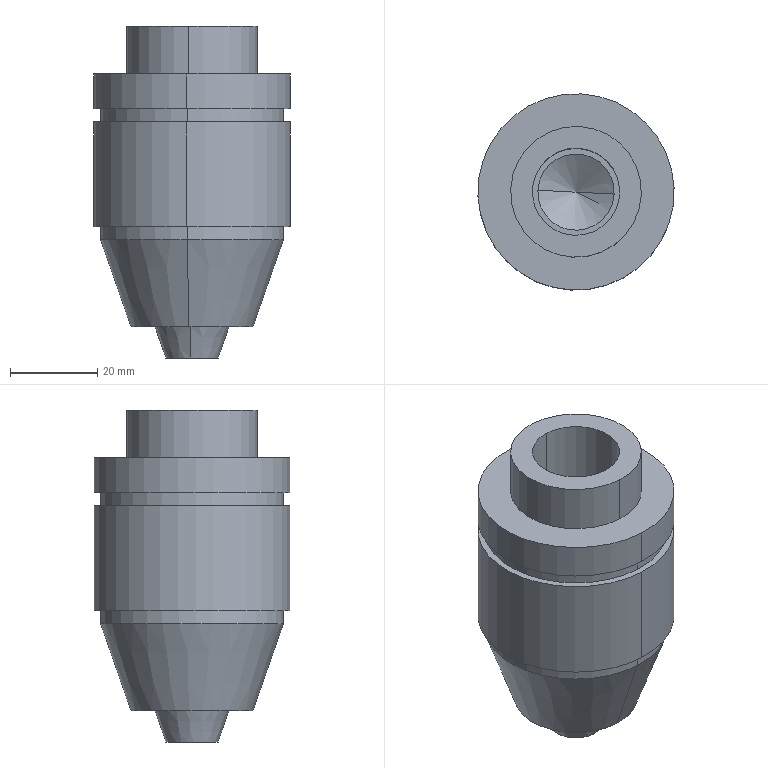Component | SolidWorks | 13-1 | 1 solid | 28 faces | box 45 x 45 x 76.14 mm | volume 73334 mm3 | cylinder 14 | plane 8 | cone 6 | commonest cylinder face diameters 42 x4 45 x4 17.5 x2 20 x2 30 x2
build123d program:
from build123d import *

# Parameters (mm, degrees)
M20_TAPPED_HOLE1_D     = 17.5
M20_TAPPED_HOLE1_DEPTH = 45
M20_TAPPED_HOLE1_TIP   = 5.258
SKETCH1_R              = 10
CUT_EXTRUDE1_DEPTH     = 42


with BuildPart() as part:
    # Sketch1_2 → Revolve1 (revolve)
    with BuildSketch(Plane.XY):
        Polygon((0, 0), (15, 0), (15, -11), (22.5, -11), (22.5, -19), (21, -19), (21, -22), (22.5, -22), (22.5, -46), (21, -46), (21, -49), (14, -69), (8.5, -69), (6, -76.143), (0, -76.143), align=None)
    revolve(axis=Axis((0, -76.143, 0), (0, 1, 0)))

    # M20 Tapped Hole1
    with Locations(Plane(origin=(0, 0, 0), x_dir=(1, 0, 0), z_dir=(0, 1, 0))):
        with Locations((0, 0)):
            Hole(M20_TAPPED_HOLE1_D / 2, depth=M20_TAPPED_HOLE1_DEPTH)
            with Locations((0, 0, -(M20_TAPPED_HOLE1_DEPTH + M20_TAPPED_HOLE1_TIP / 2))):  # 118° drill point
                Cone(0, M20_TAPPED_HOLE1_D / 2, M20_TAPPED_HOLE1_TIP, mode=Mode.SUBTRACT)

    # Sketch1 → Cut-Extrude1 (cut)
    with BuildSketch(Plane(origin=(0, 0, 0), x_dir=(1, 0, 0), z_dir=(0, 1, 0))):
        with Locations(Location((0, 0, 0), (0, 0, 180))):
            Circle(SKETCH1_R)
    extrude(amount=-CUT_EXTRUDE1_DEPTH, mode=Mode.SUBTRACT)


solid = part.part

# Placed as in the assembly
solid = solid.moved(Location((-135.043, 380.991, 535.213), (90, 0, 0)))
STEP:
#1=COLOUR_RGB('',0.7922,0.8196,0.9333);
#2=FILL_AREA_STYLE_COLOUR('',#1);
#3=FILL_AREA_STYLE('',(#2));
#4=SURFACE_STYLE_FILL_AREA(#3);
#5=SURFACE_SIDE_STYLE('',(#4));
#6=SURFACE_STYLE_USAGE(.BOTH.,#5);
#7=PRESENTATION_STYLE_ASSIGNMENT((#6));
#8=CARTESIAN_POINT('',(-5.661,15.017,19.3));
#9=VERTEX_POINT('',#8);
#10=CARTESIAN_POINT('',(-4.973,14.982,19.3));
#11=VERTEX_POINT('',#10);
#12=CARTESIAN_POINT('',(-5.317,15.,19.3));
#13=DIRECTION('',(-0.,0.,1.));
#14=DIRECTION('',(0.9987,-0.05151,0.));
#15=AXIS2_PLACEMENT_3D('',#12,#13,#14);
#16=CIRCLE('',#15,0.3445);
#17=EDGE_CURVE('',#9,#11,#16,.T.);
#18=ORIENTED_EDGE('',*,*,#17,.F.);
#19=CARTESIAN_POINT('',(-5.661,15.017,19.418));
#20=VERTEX_POINT('',#19);
#21=CARTESIAN_POINT('',(-5.661,15.017,21.071));
#22=DIRECTION('',(-0.,0.,1.));
#23=VECTOR('',#22,39.37);
#24=LINE('',#21,#23);
#25=EDGE_CURVE('',#9,#20,#24,.T.);
#26=ORIENTED_EDGE('',*,*,#25,.T.);
#27=CARTESIAN_POINT('',(-4.973,14.982,19.418));
#28=VERTEX_POINT('',#27);
#29=CARTESIAN_POINT('',(-5.317,15.,19.418));
#30=DIRECTION('',(0.,-0.,-1.));
#31=DIRECTION('',(-0.05151,-0.9987,0.));
#32=AXIS2_PLACEMENT_3D('',#29,#30,#31);
#33=CIRCLE('',#32,0.3445);
#34=EDGE_CURVE('',#28,#20,#33,.T.);
#35=ORIENTED_EDGE('',*,*,#34,.F.);
#36=CARTESIAN_POINT('',(-4.973,14.982,21.071));
#37=DIRECTION('',(-0.,0.,1.));
#38=VECTOR('',#37,39.37);
#39=LINE('',#36,#38);
#40=EDGE_CURVE('',#11,#28,#39,.T.);
#41=ORIENTED_EDGE('',*,*,#40,.F.);
#42=EDGE_LOOP('',(#18,#26,#35,#41));
#43=FACE_OUTER_BOUND('',#42,.T.);
#44=CARTESIAN_POINT('',(-5.317,15.,21.071));
#45=DIRECTION('',(-0.,0.,1.));
#46=DIRECTION('',(0.9987,-0.05151,0.));
#47=AXIS2_PLACEMENT_3D('',#44,#45,#46);
#48=CYLINDRICAL_SURFACE('',#47,0.3445);
#49=ADVANCED_FACE('',(#43),#48,.F.);
#50=CARTESIAN_POINT('',(-5.317,15.,19.093));
#51=VERTEX_POINT('',#50);
#52=CARTESIAN_POINT('',(-4.973,14.982,19.3));
#53=DIRECTION('',(0.856,-0.04415,0.515));
#54=VECTOR('',#53,39.37);
#55=LINE('',#52,#54);
#56=EDGE_CURVE('',#51,#11,#55,.T.);
#57=ORIENTED_EDGE('',*,*,#56,.F.);
#58=CARTESIAN_POINT('',(-5.661,15.017,19.3));
#59=DIRECTION('',(-0.856,0.04415,0.515));
#60=VECTOR('',#59,39.37);
#61=LINE('',#58,#60);
#62=EDGE_CURVE('',#51,#9,#61,.T.);
#63=ORIENTED_EDGE('',*,*,#62,.T.);
#64=ORIENTED_EDGE('',*,*,#17,.T.);
#65=EDGE_LOOP('',(#57,#63,#64));
#66=FACE_OUTER_BOUND('',#65,.T.);
#67=CARTESIAN_POINT('',(-5.317,15.,19.3));
#68=DIRECTION('',(-0.,0.,1.));
#69=DIRECTION('',(0.9987,-0.05151,0.));
#70=AXIS2_PLACEMENT_3D('',#67,#68,#69);
#71=CONICAL_SURFACE('',#70,0.3445,1.03);
#72=ADVANCED_FACE('',(#66),#71,.F.);
#73=CARTESIAN_POINT('',(-5.296,15.393,19.418));
#74=VERTEX_POINT('',#73);
#75=CARTESIAN_POINT('',(-5.337,14.606,19.418));
#76=VERTEX_POINT('',#75);
#77=CARTESIAN_POINT('',(-5.317,15.,19.418));
#78=DIRECTION('',(-0.,0.,1.));
#79=DIRECTION('',(-0.05151,-0.9987,0.));
#80=AXIS2_PLACEMENT_3D('',#77,#78,#79);
#81=CIRCLE('',#80,0.3937);
#82=EDGE_CURVE('',#74,#76,#81,.T.);
#83=ORIENTED_EDGE('',*,*,#82,.F.);
#84=CARTESIAN_POINT('',(-5.296,15.393,21.071));
#85=VERTEX_POINT('',#84);
#86=CARTESIAN_POINT('',(-5.296,15.393,19.418));
#87=DIRECTION('',(-0.,0.,1.));
#88=VECTOR('',#87,39.37);
#89=LINE('',#86,#88);
#90=EDGE_CURVE('',#74,#85,#89,.T.);
#91=ORIENTED_EDGE('',*,*,#90,.T.);
#92=CARTESIAN_POINT('',(-5.337,14.606,21.071));
#93=VERTEX_POINT('',#92);
#94=CARTESIAN_POINT('',(-5.317,15.,21.071));
#95=DIRECTION('',(-0.,0.,1.));
#96=DIRECTION('',(-0.05151,-0.9987,0.));
#97=AXIS2_PLACEMENT_3D('',#94,#95,#96);
#98=CIRCLE('',#97,0.3937);
#99=EDGE_CURVE('',#85,#93,#98,.T.);
#100=ORIENTED_EDGE('',*,*,#99,.T.);
#101=CARTESIAN_POINT('',(-5.337,14.606,19.418));
#102=DIRECTION('',(-0.,0.,1.));
#103=VECTOR('',#102,39.37);
#104=LINE('',#101,#103);
#105=EDGE_CURVE('',#76,#93,#104,.T.);
#106=ORIENTED_EDGE('',*,*,#105,.F.);
#107=EDGE_LOOP('',(#83,#91,#100,#106));
#108=FACE_OUTER_BOUND('',#107,.T.);
#109=CARTESIAN_POINT('',(-5.317,15.,19.418));
#110=DIRECTION('',(-0.,0.,1.));
#111=DIRECTION('',(-0.05151,-0.9987,0.));
#112=AXIS2_PLACEMENT_3D('',#109,#110,#111);
#113=CYLINDRICAL_SURFACE('',#112,0.3937);
#114=ADVANCED_FACE('',(#108),#113,.F.);
#115=CARTESIAN_POINT('',(-5.304,15.236,18.074));
#116=VERTEX_POINT('',#115);
#117=CARTESIAN_POINT('',(-5.329,14.764,18.074));
#118=VERTEX_POINT('',#117);
#119=CARTESIAN_POINT('',(-5.317,15.,18.074));
#120=DIRECTION('',(0.,-0.,-1.));
#121=DIRECTION('',(0.05151,0.9987,0.));
#122=AXIS2_PLACEMENT_3D('',#119,#120,#121);
#123=CIRCLE('',#122,0.2362);
#124=EDGE_CURVE('',#116,#118,#123,.T.);
#125=ORIENTED_EDGE('',*,*,#124,.F.);
#126=CARTESIAN_POINT('',(-5.299,15.334,18.355));
#127=VERTEX_POINT('',#126);
#128=CARTESIAN_POINT('',(-5.304,15.236,18.074));
#129=DIRECTION('',(0.01702,0.3299,0.9439));
#130=VECTOR('',#129,39.37);
#131=LINE('',#128,#130);
#132=EDGE_CURVE('',#116,#127,#131,.T.);
#133=ORIENTED_EDGE('',*,*,#132,.T.);
#134=CARTESIAN_POINT('',(-5.334,14.665,18.355));
#135=VERTEX_POINT('',#134);
#136=CARTESIAN_POINT('',(-5.317,15.,18.355));
#137=DIRECTION('',(0.,-0.,-1.));
#138=DIRECTION('',(0.05151,0.9987,0.));
#139=AXIS2_PLACEMENT_3D('',#136,#137,#138);
#140=CIRCLE('',#139,0.3346);
#141=EDGE_CURVE('',#127,#135,#140,.T.);
#142=ORIENTED_EDGE('',*,*,#141,.T.);
#143=CARTESIAN_POINT('',(-5.329,14.764,18.074));
#144=DIRECTION('',(-0.01702,-0.3299,0.9439));
#145=VECTOR('',#144,39.37);
#146=LINE('',#143,#145);
#147=EDGE_CURVE('',#118,#135,#146,.T.);
#148=ORIENTED_EDGE('',*,*,#147,.F.);
#149=EDGE_LOOP('',(#125,#133,#142,#148));
#150=FACE_OUTER_BOUND('',#149,.T.);
#151=CARTESIAN_POINT('',(-5.317,15.,18.074));
#152=DIRECTION('',(-0.,0.,1.));
#153=DIRECTION('',(-0.05151,-0.9987,0.));
#154=AXIS2_PLACEMENT_3D('',#151,#152,#153);
#155=CONICAL_SURFACE('',#154,0.2362,0.3367);
#156=ADVANCED_FACE('',(#150),#155,.T.);
#157=CARTESIAN_POINT('',(-5.288,15.55,18.355));
#158=VERTEX_POINT('',#157);
#159=CARTESIAN_POINT('',(-5.345,14.449,18.355));
#160=VERTEX_POINT('',#159);
#161=CARTESIAN_POINT('',(-5.317,15.,18.355));
#162=DIRECTION('',(0.,-0.,-1.));
#163=DIRECTION('',(0.05151,0.9987,0.));
#164=AXIS2_PLACEMENT_3D('',#161,#162,#163);
#165=CIRCLE('',#164,0.5512);
#166=EDGE_CURVE('',#158,#160,#165,.T.);
#167=ORIENTED_EDGE('',*,*,#166,.F.);
#168=CARTESIAN_POINT('',(-5.274,15.825,19.142));
#169=VERTEX_POINT('',#168);
#170=CARTESIAN_POINT('',(-5.288,15.55,18.355));
#171=DIRECTION('',(0.01702,0.3299,0.9439));
#172=VECTOR('',#171,39.37);
#173=LINE('',#170,#172);
#174=EDGE_CURVE('',#158,#169,#173,.T.);
#175=ORIENTED_EDGE('',*,*,#174,.T.);
#176=CARTESIAN_POINT('',(-5.359,14.174,19.142));
#177=VERTEX_POINT('',#176);
#178=CARTESIAN_POINT('',(-5.317,15.,19.142));
#179=DIRECTION('',(0.,-0.,-1.));
#180=DIRECTION('',(0.05151,0.9987,-0.));
#181=AXIS2_PLACEMENT_3D('',#178,#179,#180);
#182=CIRCLE('',#181,0.8268);
#183=EDGE_CURVE('',#169,#177,#182,.T.);
#184=ORIENTED_EDGE('',*,*,#183,.T.);
#185=CARTESIAN_POINT('',(-5.345,14.449,18.355));
#186=DIRECTION('',(-0.01702,-0.3299,0.9439));
#187=VECTOR('',#186,39.37);
#188=LINE('',#185,#187);
#189=EDGE_CURVE('',#160,#177,#188,.T.);
#190=ORIENTED_EDGE('',*,*,#189,.F.);
#191=EDGE_LOOP('',(#167,#175,#184,#190));
#192=FACE_OUTER_BOUND('',#191,.T.);
#193=CARTESIAN_POINT('',(-5.317,15.,18.355));
#194=DIRECTION('',(-0.,0.,1.));
#195=DIRECTION('',(-0.05151,-0.9987,0.));
#196=AXIS2_PLACEMENT_3D('',#193,#194,#195);
#197=CONICAL_SURFACE('',#196,0.5512,0.3367);
#198=ADVANCED_FACE('',(#192),#197,.T.);
#199=CARTESIAN_POINT('',(-5.274,15.825,19.26));
#200=VERTEX_POINT('',#199);
#201=CARTESIAN_POINT('',(-5.359,14.174,19.26));
#202=VERTEX_POINT('',#201);
#203=CARTESIAN_POINT('',(-5.317,15.,19.26));
#204=DIRECTION('',(0.,-0.,-1.));
#205=DIRECTION('',(0.05151,0.9987,-0.));
#206=AXIS2_PLACEMENT_3D('',#203,#204,#205);
#207=CIRCLE('',#206,0.8268);
#208=EDGE_CURVE('',#200,#202,#207,.T.);
#209=ORIENTED_EDGE('',*,*,#208,.T.);
#210=CARTESIAN_POINT('',(-5.359,14.174,18.074));
#211=DIRECTION('',(0.,-0.,-1.));
#212=VECTOR('',#211,39.37);
#213=LINE('',#210,#212);
#214=EDGE_CURVE('',#202,#177,#213,.T.);
#215=ORIENTED_EDGE('',*,*,#214,.T.);
#216=ORIENTED_EDGE('',*,*,#183,.F.);
#217=CARTESIAN_POINT('',(-5.274,15.825,18.074));
#218=DIRECTION('',(0.,-0.,-1.));
#219=VECTOR('',#218,39.37);
#220=LINE('',#217,#219);
#221=EDGE_CURVE('',#200,#169,#220,.T.);
#222=ORIENTED_EDGE('',*,*,#221,.F.);
#223=EDGE_LOOP('',(#209,#215,#216,#222));
#224=FACE_OUTER_BOUND('',#223,.T.);
#225=CARTESIAN_POINT('',(-5.317,15.,18.074));
#226=DIRECTION('',(0.,-0.,-1.));
#227=DIRECTION('',(0.05151,0.9987,-0.));
#228=AXIS2_PLACEMENT_3D('',#225,#226,#227);
#229=CYLINDRICAL_SURFACE('',#228,0.8268);
#230=ADVANCED_FACE('',(#224),#229,.T.);
#231=CARTESIAN_POINT('',(-5.271,15.884,20.205));
#232=VERTEX_POINT('',#231);
#233=CARTESIAN_POINT('',(-5.362,14.115,20.205));
#234=VERTEX_POINT('',#233);
#235=CARTESIAN_POINT('',(-5.317,15.,20.205));
#236=DIRECTION('',(0.,-0.,-1.));
#237=DIRECTION('',(0.05151,0.9987,0.));
#238=AXIS2_PLACEMENT_3D('',#235,#236,#237);
#239=CIRCLE('',#238,0.8858);
#240=EDGE_CURVE('',#232,#234,#239,.T.);
#241=ORIENTED_EDGE('',*,*,#240,.T.);
#242=CARTESIAN_POINT('',(-5.362,14.115,19.26));
#243=VERTEX_POINT('',#242);
#244=CARTESIAN_POINT('',(-5.362,14.115,18.074));
#245=DIRECTION('',(0.,-0.,-1.));
#246=VECTOR('',#245,39.37);
#247=LINE('',#244,#246);
#248=EDGE_CURVE('',#234,#243,#247,.T.);
#249=ORIENTED_EDGE('',*,*,#248,.T.);
#250=CARTESIAN_POINT('',(-5.271,15.884,19.26));
#251=VERTEX_POINT('',#250);
#252=CARTESIAN_POINT('',(-5.317,15.,19.26));
#253=DIRECTION('',(0.,-0.,-1.));
#254=DIRECTION('',(0.05151,0.9987,-0.));
#255=AXIS2_PLACEMENT_3D('',#252,#253,#254);
#256=CIRCLE('',#255,0.8858);
#257=EDGE_CURVE('',#251,#243,#256,.T.);
#258=ORIENTED_EDGE('',*,*,#257,.F.);
#259=CARTESIAN_POINT('',(-5.271,15.884,18.074));
#260=DIRECTION('',(0.,-0.,-1.));
#261=VECTOR('',#260,39.37);
#262=LINE('',#259,#261);
#263=EDGE_CURVE('',#232,#251,#262,.T.);
#264=ORIENTED_EDGE('',*,*,#263,.F.);
#265=EDGE_LOOP('',(#241,#249,#258,#264));
#266=FACE_OUTER_BOUND('',#265,.T.);
#267=CARTESIAN_POINT('',(-5.317,15.,18.074));
#268=DIRECTION('',(0.,-0.,-1.));
#269=DIRECTION('',(0.05151,0.9987,-0.));
#270=AXIS2_PLACEMENT_3D('',#267,#268,#269);
#271=CYLINDRICAL_SURFACE('',#270,0.8858);
#272=ADVANCED_FACE('',(#266),#271,.T.);
#273=CARTESIAN_POINT('',(-5.274,15.825,20.323));
#274=VERTEX_POINT('',#273);
#275=CARTESIAN_POINT('',(-5.359,14.174,20.323));
#276=VERTEX_POINT('',#275);
#277=CARTESIAN_POINT('',(-5.317,15.,20.323));
#278=DIRECTION('',(0.,-0.,-1.));
#279=DIRECTION('',(0.05151,0.9987,0.));
#280=AXIS2_PLACEMENT_3D('',#277,#278,#279);
#281=CIRCLE('',#280,0.8268);
#282=EDGE_CURVE('',#274,#276,#281,.T.);
#283=ORIENTED_EDGE('',*,*,#282,.T.);
#284=CARTESIAN_POINT('',(-5.359,14.174,20.205));
#285=VERTEX_POINT('',#284);
#286=CARTESIAN_POINT('',(-5.359,14.174,18.074));
#287=DIRECTION('',(0.,-0.,-1.));
#288=VECTOR('',#287,39.37);
#289=LINE('',#286,#288);
#290=EDGE_CURVE('',#276,#285,#289,.T.);
#291=ORIENTED_EDGE('',*,*,#290,.T.);
#292=CARTESIAN_POINT('',(-5.274,15.825,20.205));
#293=VERTEX_POINT('',#292);
#294=CARTESIAN_POINT('',(-5.317,15.,20.205));
#295=DIRECTION('',(0.,-0.,-1.));
#296=DIRECTION('',(0.05151,0.9987,0.));
#297=AXIS2_PLACEMENT_3D('',#294,#295,#296);
#298=CIRCLE('',#297,0.8268);
#299=EDGE_CURVE('',#293,#285,#298,.T.);
#300=ORIENTED_EDGE('',*,*,#299,.F.);
#301=CARTESIAN_POINT('',(-5.274,15.825,18.074));
#302=DIRECTION('',(0.,-0.,-1.));
#303=VECTOR('',#302,39.37);
#304=LINE('',#301,#303);
#305=EDGE_CURVE('',#274,#293,#304,.T.);
#306=ORIENTED_EDGE('',*,*,#305,.F.);
#307=EDGE_LOOP('',(#283,#291,#300,#306));
#308=FACE_OUTER_BOUND('',#307,.T.);
#309=CARTESIAN_POINT('',(-5.317,15.,18.074));
#310=DIRECTION('',(0.,-0.,-1.));
#311=DIRECTION('',(0.05151,0.9987,-0.));
#312=AXIS2_PLACEMENT_3D('',#309,#310,#311);
#313=CYLINDRICAL_SURFACE('',#312,0.8268);
#314=ADVANCED_FACE('',(#308),#313,.T.);
#315=CARTESIAN_POINT('',(-5.271,15.884,20.638));
#316=VERTEX_POINT('',#315);
#317=CARTESIAN_POINT('',(-5.362,14.115,20.638));
#318=VERTEX_POINT('',#317);
#319=CARTESIAN_POINT('',(-5.317,15.,20.638));
#320=DIRECTION('',(0.,-0.,-1.));
#321=DIRECTION('',(0.05151,0.9987,0.));
#322=AXIS2_PLACEMENT_3D('',#319,#320,#321);
#323=CIRCLE('',#322,0.8858);
#324=EDGE_CURVE('',#316,#318,#323,.T.);
#325=ORIENTED_EDGE('',*,*,#324,.T.);
#326=CARTESIAN_POINT('',(-5.362,14.115,20.323));
#327=VERTEX_POINT('',#326);
#328=CARTESIAN_POINT('',(-5.362,14.115,18.074));
#329=DIRECTION('',(0.,-0.,-1.));
#330=VECTOR('',#329,39.37);
#331=LINE('',#328,#330);
#332=EDGE_CURVE('',#318,#327,#331,.T.);
#333=ORIENTED_EDGE('',*,*,#332,.T.);
#334=CARTESIAN_POINT('',(-5.271,15.884,20.323));
#335=VERTEX_POINT('',#334);
#336=CARTESIAN_POINT('',(-5.317,15.,20.323));
#337=DIRECTION('',(0.,-0.,-1.));
#338=DIRECTION('',(0.05151,0.9987,0.));
#339=AXIS2_PLACEMENT_3D('',#336,#337,#338);
#340=CIRCLE('',#339,0.8858);
#341=EDGE_CURVE('',#335,#327,#340,.T.);
#342=ORIENTED_EDGE('',*,*,#341,.F.);
#343=CARTESIAN_POINT('',(-5.271,15.884,18.074));
#344=DIRECTION('',(0.,-0.,-1.));
#345=VECTOR('',#344,39.37);
#346=LINE('',#343,#345);
#347=EDGE_CURVE('',#316,#335,#346,.T.);
#348=ORIENTED_EDGE('',*,*,#347,.F.);
#349=EDGE_LOOP('',(#325,#333,#342,#348));
#350=FACE_OUTER_BOUND('',#349,.T.);
#351=CARTESIAN_POINT('',(-5.317,15.,18.074));
#352=DIRECTION('',(0.,-0.,-1.));
#353=DIRECTION('',(0.05151,0.9987,-0.));
#354=AXIS2_PLACEMENT_3D('',#351,#352,#353);
#355=CYLINDRICAL_SURFACE('',#354,0.8858);
#356=ADVANCED_FACE('',(#350),#355,.T.);
#357=CARTESIAN_POINT('',(-5.286,15.589,21.071));
#358=VERTEX_POINT('',#357);
#359=CARTESIAN_POINT('',(-5.347,14.41,21.071));
#360=VERTEX_POINT('',#359);
#361=CARTESIAN_POINT('',(-5.317,15.,21.071));
#362=DIRECTION('',(0.,-0.,-1.));
#363=DIRECTION('',(0.05151,0.9987,0.));
#364=AXIS2_PLACEMENT_3D('',#361,#362,#363);
#365=CIRCLE('',#364,0.5906);
#366=EDGE_CURVE('',#358,#360,#365,.T.);
#367=ORIENTED_EDGE('',*,*,#366,.T.);
#368=CARTESIAN_POINT('',(-5.347,14.41,20.638));
#369=VERTEX_POINT('',#368);
#370=CARTESIAN_POINT('',(-5.347,14.41,18.074));
#371=DIRECTION('',(0.,-0.,-1.));
#372=VECTOR('',#371,39.37);
#373=LINE('',#370,#372);
#374=EDGE_CURVE('',#360,#369,#373,.T.);
#375=ORIENTED_EDGE('',*,*,#374,.T.);
#376=CARTESIAN_POINT('',(-5.286,15.589,20.638));
#377=VERTEX_POINT('',#376);
#378=CARTESIAN_POINT('',(-5.317,15.,20.638));
#379=DIRECTION('',(0.,-0.,-1.));
#380=DIRECTION('',(0.05151,0.9987,0.));
#381=AXIS2_PLACEMENT_3D('',#378,#379,#380);
#382=CIRCLE('',#381,0.5906);
#383=EDGE_CURVE('',#377,#369,#382,.T.);
#384=ORIENTED_EDGE('',*,*,#383,.F.);
#385=CARTESIAN_POINT('',(-5.286,15.589,18.074));
#386=DIRECTION('',(0.,-0.,-1.));
#387=VECTOR('',#386,39.37);
#388=LINE('',#385,#387);
#389=EDGE_CURVE('',#358,#377,#388,.T.);
#390=ORIENTED_EDGE('',*,*,#389,.F.);
#391=EDGE_LOOP('',(#367,#375,#384,#390));
#392=FACE_OUTER_BOUND('',#391,.T.);
#393=CARTESIAN_POINT('',(-5.317,15.,18.074));
#394=DIRECTION('',(0.,-0.,-1.));
#395=DIRECTION('',(0.05151,0.9987,0.));
#396=AXIS2_PLACEMENT_3D('',#393,#394,#395);
#397=CYLINDRICAL_SURFACE('',#396,0.5906);
#398=ADVANCED_FACE('',(#392),#397,.T.);
#399=CARTESIAN_POINT('',(-5.317,15.,21.071));
#400=DIRECTION('',(-0.,0.,1.));
#401=DIRECTION('',(-0.05151,-0.9987,0.));
#402=AXIS2_PLACEMENT_3D('',#399,#400,#401);
#403=CIRCLE('',#402,0.3937);
#404=EDGE_CURVE('',#93,#85,#403,.T.);
#405=ORIENTED_EDGE('',*,*,#404,.F.);
#406=ORIENTED_EDGE('',*,*,#99,.F.);
#407=EDGE_LOOP('',(#405,#406));
#408=FACE_BOUND('',#407,.T.);
#409=ORIENTED_EDGE('',*,*,#366,.F.);
#410=CARTESIAN_POINT('',(-5.317,15.,21.071));
#411=DIRECTION('',(0.,-0.,-1.));
#412=DIRECTION('',(0.05151,0.9987,0.));
#413=AXIS2_PLACEMENT_3D('',#410,#411,#412);
#414=CIRCLE('',#413,0.5906);
#415=EDGE_CURVE('',#360,#358,#414,.T.);
#416=ORIENTED_EDGE('',*,*,#415,.F.);
#417=EDGE_LOOP('',(#409,#416));
#418=FACE_OUTER_BOUND('',#417,.T.);
#419=CARTESIAN_POINT('',(-5.317,15.,21.071));
#420=DIRECTION('',(-0.,0.,1.));
#421=DIRECTION('',(-0.05151,-0.9987,0.));
#422=AXIS2_PLACEMENT_3D('',#419,#420,#421);
#423=PLANE('',#422);
#424=ADVANCED_FACE('',(#408,#418),#423,.T.);
#425=ORIENTED_EDGE('',*,*,#374,.F.);
#426=ORIENTED_EDGE('',*,*,#415,.T.);
#427=ORIENTED_EDGE('',*,*,#389,.T.);
#428=CARTESIAN_POINT('',(-5.317,15.,20.638));
#429=DIRECTION('',(0.,-0.,-1.));
#430=DIRECTION('',(0.05151,0.9987,0.));
#431=AXIS2_PLACEMENT_3D('',#428,#429,#430);
#432=CIRCLE('',#431,0.5906);
#433=EDGE_CURVE('',#369,#377,#432,.T.);
#434=ORIENTED_EDGE('',*,*,#433,.F.);
#435=EDGE_LOOP('',(#425,#426,#427,#434));
#436=FACE_OUTER_BOUND('',#435,.T.);
#437=CARTESIAN_POINT('',(-5.317,15.,18.074));
#438=DIRECTION('',(0.,-0.,-1.));
#439=DIRECTION('',(0.05151,0.9987,0.));
#440=AXIS2_PLACEMENT_3D('',#437,#438,#439);
#441=CYLINDRICAL_SURFACE('',#440,0.5906);
#442=ADVANCED_FACE('',(#436),#441,.T.);
#443=ORIENTED_EDGE('',*,*,#383,.T.);
#444=ORIENTED_EDGE('',*,*,#433,.T.);
#445=EDGE_LOOP('',(#443,#444));
#446=FACE_BOUND('',#445,.T.);
#447=ORIENTED_EDGE('',*,*,#324,.F.);
#448=CARTESIAN_POINT('',(-5.317,15.,20.638));
#449=DIRECTION('',(0.,-0.,-1.));
#450=DIRECTION('',(0.05151,0.9987,0.));
#451=AXIS2_PLACEMENT_3D('',#448,#449,#450);
#452=CIRCLE('',#451,0.8858);
#453=EDGE_CURVE('',#318,#316,#452,.T.);
#454=ORIENTED_EDGE('',*,*,#453,.F.);
#455=EDGE_LOOP('',(#447,#454));
#456=FACE_OUTER_BOUND('',#455,.T.);
#457=CARTESIAN_POINT('',(-5.286,15.589,20.638));
#458=DIRECTION('',(-0.,0.,1.));
#459=DIRECTION('',(-0.05151,-0.9987,0.));
#460=AXIS2_PLACEMENT_3D('',#457,#458,#459);
#461=PLANE('',#460);
#462=ADVANCED_FACE('',(#446,#456),#461,.T.);
#463=ORIENTED_EDGE('',*,*,#332,.F.);
#464=ORIENTED_EDGE('',*,*,#453,.T.);
#465=ORIENTED_EDGE('',*,*,#347,.T.);
#466=CARTESIAN_POINT('',(-5.317,15.,20.323));
#467=DIRECTION('',(0.,-0.,-1.));
#468=DIRECTION('',(0.05151,0.9987,0.));
#469=AXIS2_PLACEMENT_3D('',#466,#467,#468);
#470=CIRCLE('',#469,0.8858);
#471=EDGE_CURVE('',#327,#335,#470,.T.);
#472=ORIENTED_EDGE('',*,*,#471,.F.);
#473=EDGE_LOOP('',(#463,#464,#465,#472));
#474=FACE_OUTER_BOUND('',#473,.T.);
#475=CARTESIAN_POINT('',(-5.317,15.,18.074));
#476=DIRECTION('',(0.,-0.,-1.));
#477=DIRECTION('',(0.05151,0.9987,-0.));
#478=AXIS2_PLACEMENT_3D('',#475,#476,#477);
#479=CYLINDRICAL_SURFACE('',#478,0.8858);
#480=ADVANCED_FACE('',(#474),#479,.T.);
#481=ORIENTED_EDGE('',*,*,#341,.T.);
#482=ORIENTED_EDGE('',*,*,#471,.T.);
#483=EDGE_LOOP('',(#481,#482));
#484=FACE_OUTER_BOUND('',#483,.T.);
#485=ORIENTED_EDGE('',*,*,#282,.F.);
#486=CARTESIAN_POINT('',(-5.317,15.,20.323));
#487=DIRECTION('',(0.,-0.,-1.));
#488=DIRECTION('',(0.05151,0.9987,0.));
#489=AXIS2_PLACEMENT_3D('',#486,#487,#488);
#490=CIRCLE('',#489,0.8268);
#491=EDGE_CURVE('',#276,#274,#490,.T.);
#492=ORIENTED_EDGE('',*,*,#491,.F.);
#493=EDGE_LOOP('',(#485,#492));
#494=FACE_BOUND('',#493,.T.);
#495=CARTESIAN_POINT('',(-5.271,15.884,20.323));
#496=DIRECTION('',(0.,-0.,-1.));
#497=DIRECTION('',(0.05151,0.9987,-0.));
#498=AXIS2_PLACEMENT_3D('',#495,#496,#497);
#499=PLANE('',#498);
#500=ADVANCED_FACE('',(#484,#494),#499,.T.);
#501=ORIENTED_EDGE('',*,*,#290,.F.);
#502=ORIENTED_EDGE('',*,*,#491,.T.);
#503=ORIENTED_EDGE('',*,*,#305,.T.);
#504=CARTESIAN_POINT('',(-5.317,15.,20.205));
#505=DIRECTION('',(0.,-0.,-1.));
#506=DIRECTION('',(0.05151,0.9987,0.));
#507=AXIS2_PLACEMENT_3D('',#504,#505,#506);
#508=CIRCLE('',#507,0.8268);
#509=EDGE_CURVE('',#285,#293,#508,.T.);
#510=ORIENTED_EDGE('',*,*,#509,.F.);
#511=EDGE_LOOP('',(#501,#502,#503,#510));
#512=FACE_OUTER_BOUND('',#511,.T.);
#513=CARTESIAN_POINT('',(-5.317,15.,18.074));
#514=DIRECTION('',(0.,-0.,-1.));
#515=DIRECTION('',(0.05151,0.9987,-0.));
#516=AXIS2_PLACEMENT_3D('',#513,#514,#515);
#517=CYLINDRICAL_SURFACE('',#516,0.8268);
#518=ADVANCED_FACE('',(#512),#517,.T.);
#519=ORIENTED_EDGE('',*,*,#299,.T.);
#520=ORIENTED_EDGE('',*,*,#509,.T.);
#521=EDGE_LOOP('',(#519,#520));
#522=FACE_BOUND('',#521,.T.);
#523=ORIENTED_EDGE('',*,*,#240,.F.);
#524=CARTESIAN_POINT('',(-5.317,15.,20.205));
#525=DIRECTION('',(0.,-0.,-1.));
#526=DIRECTION('',(0.05151,0.9987,0.));
#527=AXIS2_PLACEMENT_3D('',#524,#525,#526);
#528=CIRCLE('',#527,0.8858);
#529=EDGE_CURVE('',#234,#232,#528,.T.);
#530=ORIENTED_EDGE('',*,*,#529,.F.);
#531=EDGE_LOOP('',(#523,#530));
#532=FACE_OUTER_BOUND('',#531,.T.);
#533=CARTESIAN_POINT('',(-5.274,15.825,20.205));
#534=DIRECTION('',(-0.,0.,1.));
#535=DIRECTION('',(-0.05151,-0.9987,0.));
#536=AXIS2_PLACEMENT_3D('',#533,#534,#535);
#537=PLANE('',#536);
#538=ADVANCED_FACE('',(#522,#532),#537,.T.);
#539=ORIENTED_EDGE('',*,*,#248,.F.);
#540=ORIENTED_EDGE('',*,*,#529,.T.);
#541=ORIENTED_EDGE('',*,*,#263,.T.);
#542=CARTESIAN_POINT('',(-5.317,15.,19.26));
#543=DIRECTION('',(0.,-0.,-1.));
#544=DIRECTION('',(0.05151,0.9987,-0.));
#545=AXIS2_PLACEMENT_3D('',#542,#543,#544);
#546=CIRCLE('',#545,0.8858);
#547=EDGE_CURVE('',#243,#251,#546,.T.);
#548=ORIENTED_EDGE('',*,*,#547,.F.);
#549=EDGE_LOOP('',(#539,#540,#541,#548));
#550=FACE_OUTER_BOUND('',#549,.T.);
#551=CARTESIAN_POINT('',(-5.317,15.,18.074));
#552=DIRECTION('',(0.,-0.,-1.));
#553=DIRECTION('',(0.05151,0.9987,-0.));
#554=AXIS2_PLACEMENT_3D('',#551,#552,#553);
#555=CYLINDRICAL_SURFACE('',#554,0.8858);
#556=ADVANCED_FACE('',(#550),#555,.T.);
#557=ORIENTED_EDGE('',*,*,#257,.T.);
#558=ORIENTED_EDGE('',*,*,#547,.T.);
#559=EDGE_LOOP('',(#557,#558));
#560=FACE_OUTER_BOUND('',#559,.T.);
#561=ORIENTED_EDGE('',*,*,#208,.F.);
#562=CARTESIAN_POINT('',(-5.317,15.,19.26));
#563=DIRECTION('',(0.,-0.,-1.));
#564=DIRECTION('',(0.05151,0.9987,-0.));
#565=AXIS2_PLACEMENT_3D('',#562,#563,#564);
#566=CIRCLE('',#565,0.8268);
#567=EDGE_CURVE('',#202,#200,#566,.T.);
#568=ORIENTED_EDGE('',*,*,#567,.F.);
#569=EDGE_LOOP('',(#561,#568));
#570=FACE_BOUND('',#569,.T.);
#571=CARTESIAN_POINT('',(-5.271,15.884,19.26));
#572=DIRECTION('',(0.,-0.,-1.));
#573=DIRECTION('',(0.05151,0.9987,-0.));
#574=AXIS2_PLACEMENT_3D('',#571,#572,#573);
#575=PLANE('',#574);
#576=ADVANCED_FACE('',(#560,#570),#575,.T.);
#577=ORIENTED_EDGE('',*,*,#214,.F.);
#578=ORIENTED_EDGE('',*,*,#567,.T.);
#579=ORIENTED_EDGE('',*,*,#221,.T.);
#580=CARTESIAN_POINT('',(-5.317,15.,19.142));
#581=DIRECTION('',(0.,-0.,-1.));
#582=DIRECTION('',(0.05151,0.9987,-0.));
#583=AXIS2_PLACEMENT_3D('',#580,#581,#582);
#584=CIRCLE('',#583,0.8268);
#585=EDGE_CURVE('',#177,#169,#584,.T.);
#586=ORIENTED_EDGE('',*,*,#585,.F.);
#587=EDGE_LOOP('',(#577,#578,#579,#586));
#588=FACE_OUTER_BOUND('',#587,.T.);
#589=CARTESIAN_POINT('',(-5.317,15.,18.074));
#590=DIRECTION('',(0.,-0.,-1.));
#591=DIRECTION('',(0.05151,0.9987,-0.));
#592=AXIS2_PLACEMENT_3D('',#589,#590,#591);
#593=CYLINDRICAL_SURFACE('',#592,0.8268);
#594=ADVANCED_FACE('',(#588),#593,.T.);
#595=ORIENTED_EDGE('',*,*,#174,.F.);
#596=CARTESIAN_POINT('',(-5.317,15.,18.355));
#597=DIRECTION('',(0.,-0.,-1.));
#598=DIRECTION('',(0.05151,0.9987,0.));
#599=AXIS2_PLACEMENT_3D('',#596,#597,#598);
#600=CIRCLE('',#599,0.5512);
#601=EDGE_CURVE('',#160,#158,#600,.T.);
#602=ORIENTED_EDGE('',*,*,#601,.F.);
#603=ORIENTED_EDGE('',*,*,#189,.T.);
#604=ORIENTED_EDGE('',*,*,#585,.T.);
#605=EDGE_LOOP('',(#595,#602,#603,#604));
#606=FACE_OUTER_BOUND('',#605,.T.);
#607=CARTESIAN_POINT('',(-5.317,15.,18.355));
#608=DIRECTION('',(-0.,0.,1.));
#609=DIRECTION('',(-0.05151,-0.9987,0.));
#610=AXIS2_PLACEMENT_3D('',#607,#608,#609);
#611=CONICAL_SURFACE('',#610,0.5512,0.3367);
#612=ADVANCED_FACE('',(#606),#611,.T.);
#613=ORIENTED_EDGE('',*,*,#601,.T.);
#614=ORIENTED_EDGE('',*,*,#166,.T.);
#615=EDGE_LOOP('',(#613,#614));
#616=FACE_OUTER_BOUND('',#615,.T.);
#617=CARTESIAN_POINT('',(-5.317,15.,18.355));
#618=DIRECTION('',(0.,-0.,-1.));
#619=DIRECTION('',(0.05151,0.9987,0.));
#620=AXIS2_PLACEMENT_3D('',#617,#618,#619);
#621=CIRCLE('',#620,0.3346);
#622=EDGE_CURVE('',#135,#127,#621,.T.);
#623=ORIENTED_EDGE('',*,*,#622,.F.);
#624=ORIENTED_EDGE('',*,*,#141,.F.);
#625=EDGE_LOOP('',(#623,#624));
#626=FACE_BOUND('',#625,.T.);
#627=CARTESIAN_POINT('',(-5.288,15.55,18.355));
#628=DIRECTION('',(0.,-0.,-1.));
#629=DIRECTION('',(0.05151,0.9987,-0.));
#630=AXIS2_PLACEMENT_3D('',#627,#628,#629);
#631=PLANE('',#630);
#632=ADVANCED_FACE('',(#616,#626),#631,.T.);
#633=ORIENTED_EDGE('',*,*,#132,.F.);
#634=CARTESIAN_POINT('',(-5.317,15.,18.074));
#635=DIRECTION('',(0.,-0.,-1.));
#636=DIRECTION('',(0.05151,0.9987,0.));
#637=AXIS2_PLACEMENT_3D('',#634,#635,#636);
#638=CIRCLE('',#637,0.2362);
#639=EDGE_CURVE('',#118,#116,#638,.T.);
#640=ORIENTED_EDGE('',*,*,#639,.F.);
#641=ORIENTED_EDGE('',*,*,#147,.T.);
#642=ORIENTED_EDGE('',*,*,#622,.T.);
#643=EDGE_LOOP('',(#633,#640,#641,#642));
#644=FACE_OUTER_BOUND('',#643,.T.);
#645=CARTESIAN_POINT('',(-5.317,15.,18.074));
#646=DIRECTION('',(-0.,0.,1.));
#647=DIRECTION('',(-0.05151,-0.9987,0.));
#648=AXIS2_PLACEMENT_3D('',#645,#646,#647);
#649=CONICAL_SURFACE('',#648,0.2362,0.3367);
#650=ADVANCED_FACE('',(#644),#649,.T.);
#651=ORIENTED_EDGE('',*,*,#639,.T.);
#652=ORIENTED_EDGE('',*,*,#124,.T.);
#653=EDGE_LOOP('',(#651,#652));
#654=FACE_OUTER_BOUND('',#653,.T.);
#655=CARTESIAN_POINT('',(-5.304,15.236,18.074));
#656=DIRECTION('',(0.,-0.,-1.));
#657=DIRECTION('',(0.05151,0.9987,-0.));
#658=AXIS2_PLACEMENT_3D('',#655,#656,#657);
#659=PLANE('',#658);
#660=ADVANCED_FACE('',(#654),#659,.T.);
#661=CARTESIAN_POINT('',(-5.317,15.,19.418));
#662=DIRECTION('',(-0.,0.,1.));
#663=DIRECTION('',(-0.05151,-0.9987,0.));
#664=AXIS2_PLACEMENT_3D('',#661,#662,#663);
#665=CIRCLE('',#664,0.3937);
#666=EDGE_CURVE('',#76,#74,#665,.T.);
#667=ORIENTED_EDGE('',*,*,#666,.T.);
#668=ORIENTED_EDGE('',*,*,#82,.T.);
#669=EDGE_LOOP('',(#667,#668));
#670=FACE_OUTER_BOUND('',#669,.T.);
#671=ORIENTED_EDGE('',*,*,#34,.T.);
#672=CARTESIAN_POINT('',(-5.317,15.,19.418));
#673=DIRECTION('',(0.,-0.,-1.));
#674=DIRECTION('',(-0.05151,-0.9987,0.));
#675=AXIS2_PLACEMENT_3D('',#672,#673,#674);
#676=CIRCLE('',#675,0.3445);
#677=EDGE_CURVE('',#20,#28,#676,.T.);
#678=ORIENTED_EDGE('',*,*,#677,.T.);
#679=EDGE_LOOP('',(#671,#678));
#680=FACE_BOUND('',#679,.T.);
#681=CARTESIAN_POINT('',(-5.317,15.,19.418));
#682=DIRECTION('',(-0.,0.,1.));
#683=DIRECTION('',(-0.05151,-0.9987,0.));
#684=AXIS2_PLACEMENT_3D('',#681,#682,#683);
#685=PLANE('',#684);
#686=ADVANCED_FACE('',(#670,#680),#685,.T.);
#687=ORIENTED_EDGE('',*,*,#90,.F.);
#688=ORIENTED_EDGE('',*,*,#666,.F.);
#689=ORIENTED_EDGE('',*,*,#105,.T.);
#690=ORIENTED_EDGE('',*,*,#404,.T.);
#691=EDGE_LOOP('',(#687,#688,#689,#690));
#692=FACE_OUTER_BOUND('',#691,.T.);
#693=CARTESIAN_POINT('',(-5.317,15.,19.418));
#694=DIRECTION('',(-0.,0.,1.));
#695=DIRECTION('',(-0.05151,-0.9987,0.));
#696=AXIS2_PLACEMENT_3D('',#693,#694,#695);
#697=CYLINDRICAL_SURFACE('',#696,0.3937);
#698=ADVANCED_FACE('',(#692),#697,.F.);
#699=ORIENTED_EDGE('',*,*,#62,.F.);
#700=ORIENTED_EDGE('',*,*,#56,.T.);
#701=CARTESIAN_POINT('',(-5.317,15.,19.3));
#702=DIRECTION('',(-0.,0.,1.));
#703=DIRECTION('',(0.9987,-0.05151,0.));
#704=AXIS2_PLACEMENT_3D('',#701,#702,#703);
#705=CIRCLE('',#704,0.3445);
#706=EDGE_CURVE('',#11,#9,#705,.T.);
#707=ORIENTED_EDGE('',*,*,#706,.T.);
#708=EDGE_LOOP('',(#699,#700,#707));
#709=FACE_OUTER_BOUND('',#708,.T.);
#710=CARTESIAN_POINT('',(-5.317,15.,19.3));
#711=DIRECTION('',(-0.,0.,1.));
#712=DIRECTION('',(0.9987,-0.05151,0.));
#713=AXIS2_PLACEMENT_3D('',#710,#711,#712);
#714=CONICAL_SURFACE('',#713,0.3445,1.03);
#715=ADVANCED_FACE('',(#709),#714,.F.);
#716=ORIENTED_EDGE('',*,*,#25,.F.);
#717=ORIENTED_EDGE('',*,*,#706,.F.);
#718=ORIENTED_EDGE('',*,*,#40,.T.);
#719=ORIENTED_EDGE('',*,*,#677,.F.);
#720=EDGE_LOOP('',(#716,#717,#718,#719));
#721=FACE_OUTER_BOUND('',#720,.T.);
#722=CARTESIAN_POINT('',(-5.317,15.,21.071));
#723=DIRECTION('',(-0.,0.,1.));
#724=DIRECTION('',(0.9987,-0.05151,0.));
#725=AXIS2_PLACEMENT_3D('',#722,#723,#724);
#726=CYLINDRICAL_SURFACE('',#725,0.3445);
#727=ADVANCED_FACE('',(#721),#726,.F.);
#728=CLOSED_SHELL('',(#49,#72,#114,#156,#198,#230,#272,#314,#356,#398,#424,#442,#462,#480,#500,#518,#538,#556,#576,#594,#612,#632,#650,#660,#686,#698,#715,#727));
#729=MANIFOLD_SOLID_BREP('',#728);
#730=STYLED_ITEM('',(#7),#729);
#731=PRESENTATION_LAYER_ASSIGNMENT('','',(#730));
#732=(LENGTH_UNIT()NAMED_UNIT(*)SI_UNIT($,.METRE.));
#733=LENGTH_MEASURE_WITH_UNIT(LENGTH_MEASURE(0.0254),#732);
#734=DIMENSIONAL_EXPONENTS(1.,0.,0.,0.,0.,0.,0.);
#735=(CONVERSION_BASED_UNIT('',#733)LENGTH_UNIT()NAMED_UNIT(#734));
#736=UNCERTAINTY_MEASURE_WITH_UNIT(LENGTH_MEASURE(0.00001),#735,'','');
#737=(NAMED_UNIT(*)PLANE_ANGLE_UNIT()SI_UNIT($,.RADIAN.));
#738=(NAMED_UNIT(*)SI_UNIT($,.STERADIAN.)SOLID_ANGLE_UNIT());
#739=(GEOMETRIC_REPRESENTATION_CONTEXT(3)GLOBAL_UNCERTAINTY_ASSIGNED_CONTEXT((#736))GLOBAL_UNIT_ASSIGNED_CONTEXT((#735,#737,#738))REPRESENTATION_CONTEXT('',''));
#740=MECHANICAL_DESIGN_GEOMETRIC_PRESENTATION_REPRESENTATION('',(#730),#739);
#741=CARTESIAN_POINT('',(0.,0.,0.));
#742=DIRECTION('',(0.,0.,1.));
#743=DIRECTION('',(1.,0.,0.));
#744=AXIS2_PLACEMENT_3D('',#741,#742,#743);
#745=(LENGTH_UNIT()NAMED_UNIT(*)SI_UNIT($,.METRE.));
#746=LENGTH_MEASURE_WITH_UNIT(LENGTH_MEASURE(0.0254),#745);
#747=DIMENSIONAL_EXPONENTS(1.,0.,0.,0.,0.,0.,0.);
#748=(CONVERSION_BASED_UNIT('',#746)LENGTH_UNIT()NAMED_UNIT(#747));
#749=UNCERTAINTY_MEASURE_WITH_UNIT(LENGTH_MEASURE(0.00001),#748,'','');
#750=(NAMED_UNIT(*)PLANE_ANGLE_UNIT()SI_UNIT($,.RADIAN.));
#751=(NAMED_UNIT(*)SI_UNIT($,.STERADIAN.)SOLID_ANGLE_UNIT());
#752=(GEOMETRIC_REPRESENTATION_CONTEXT(3)GLOBAL_UNCERTAINTY_ASSIGNED_CONTEXT((#749))GLOBAL_UNIT_ASSIGNED_CONTEXT((#748,#750,#751))REPRESENTATION_CONTEXT('',''));
#753=ADVANCED_BREP_SHAPE_REPRESENTATION('',(#729,#744),#752);